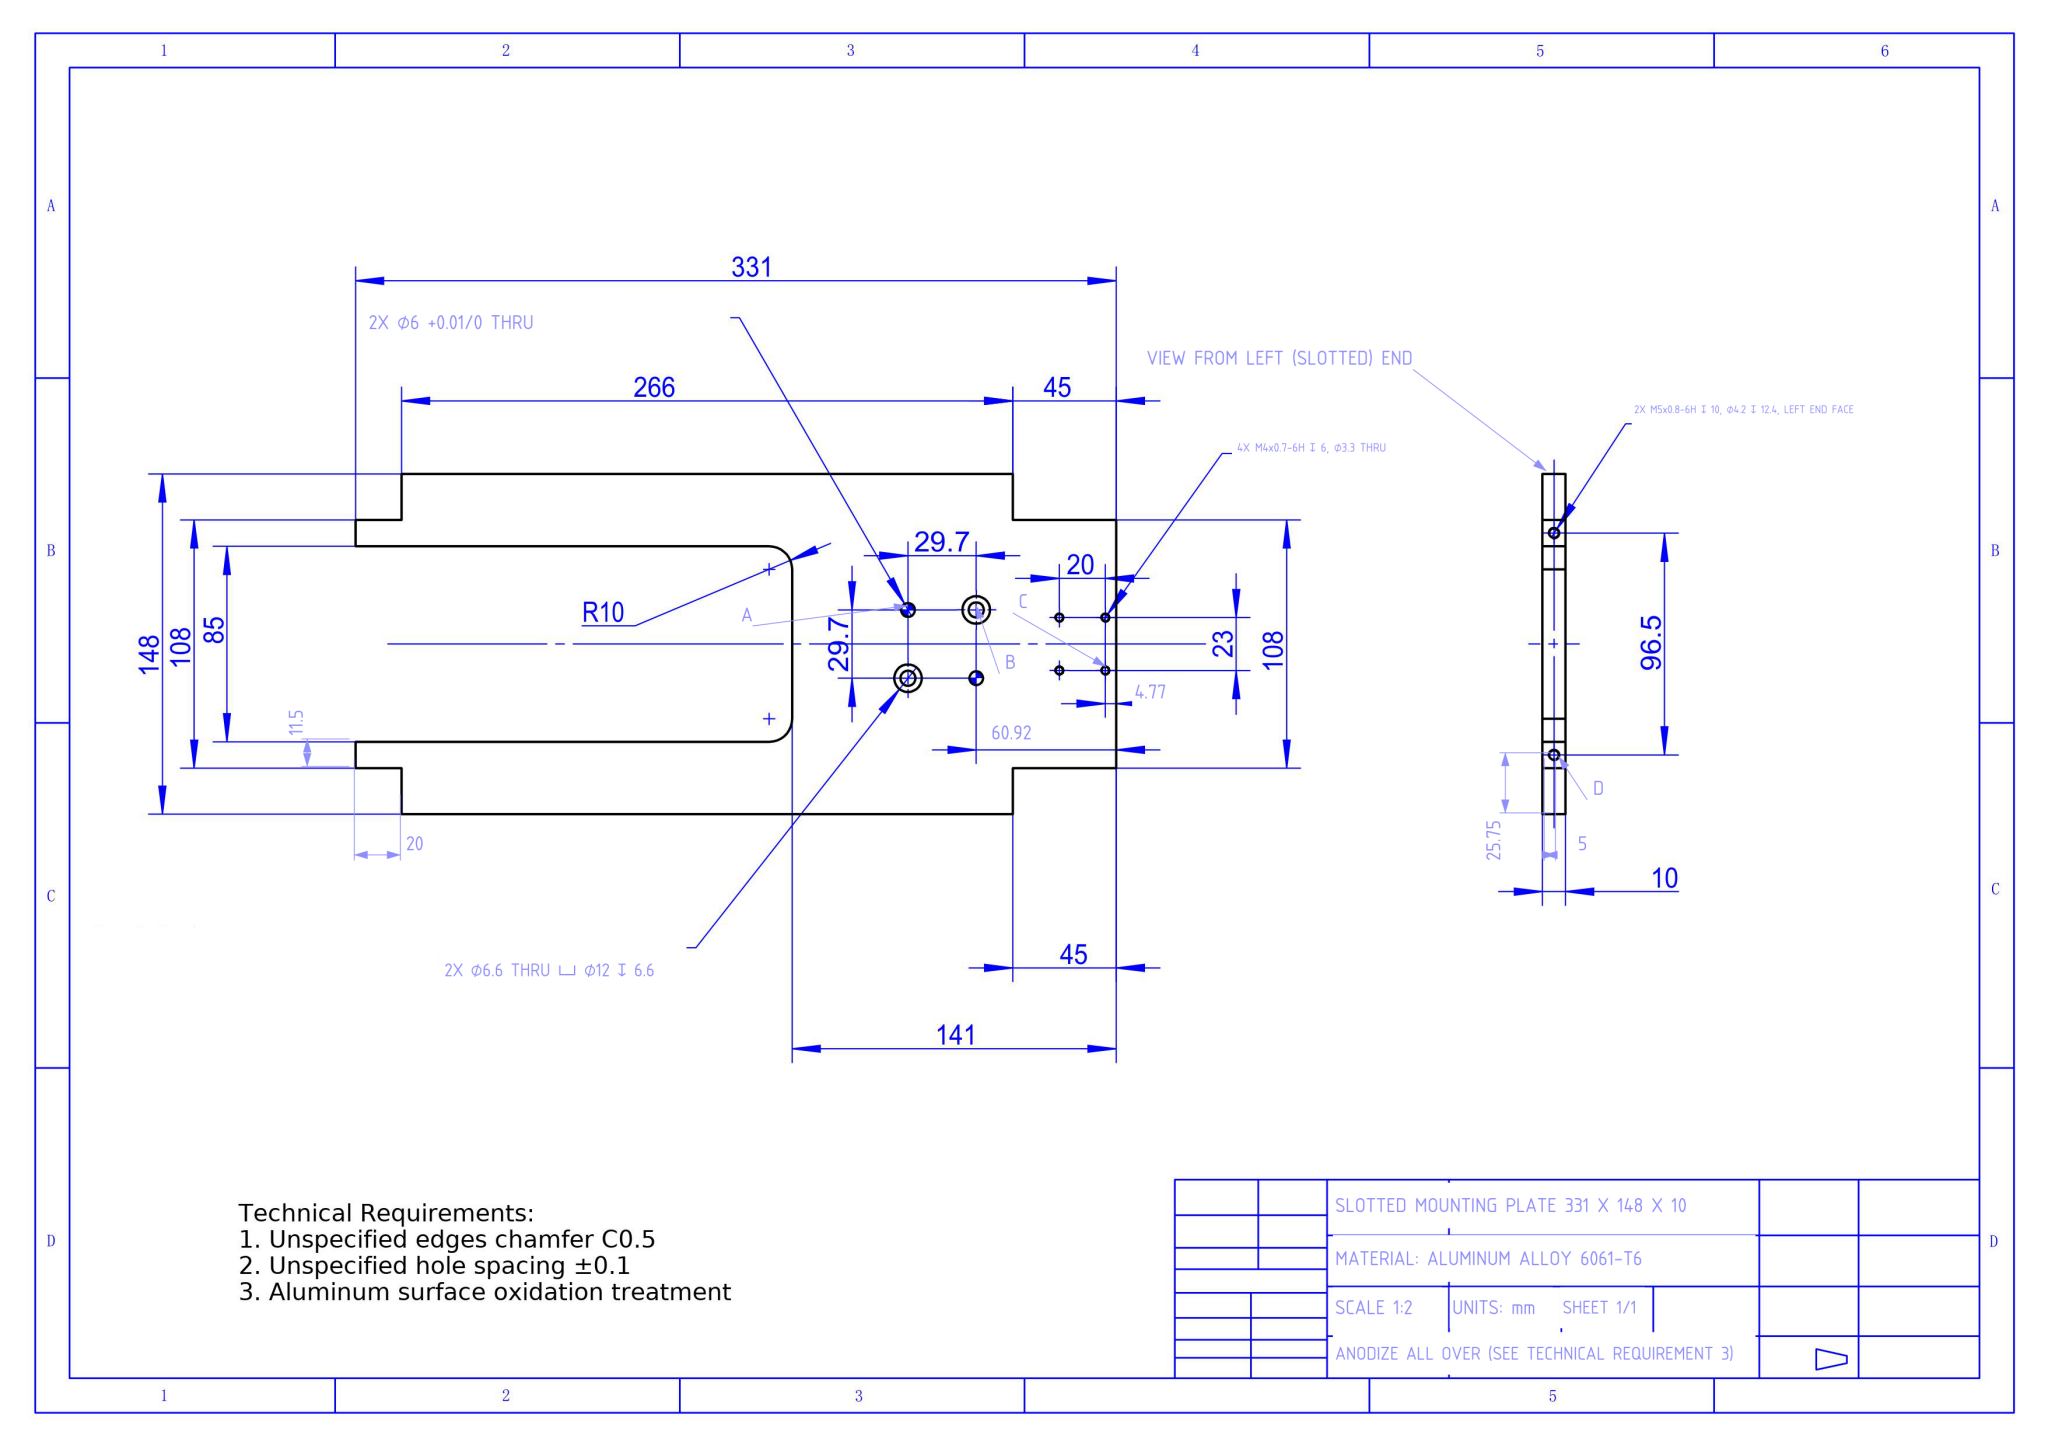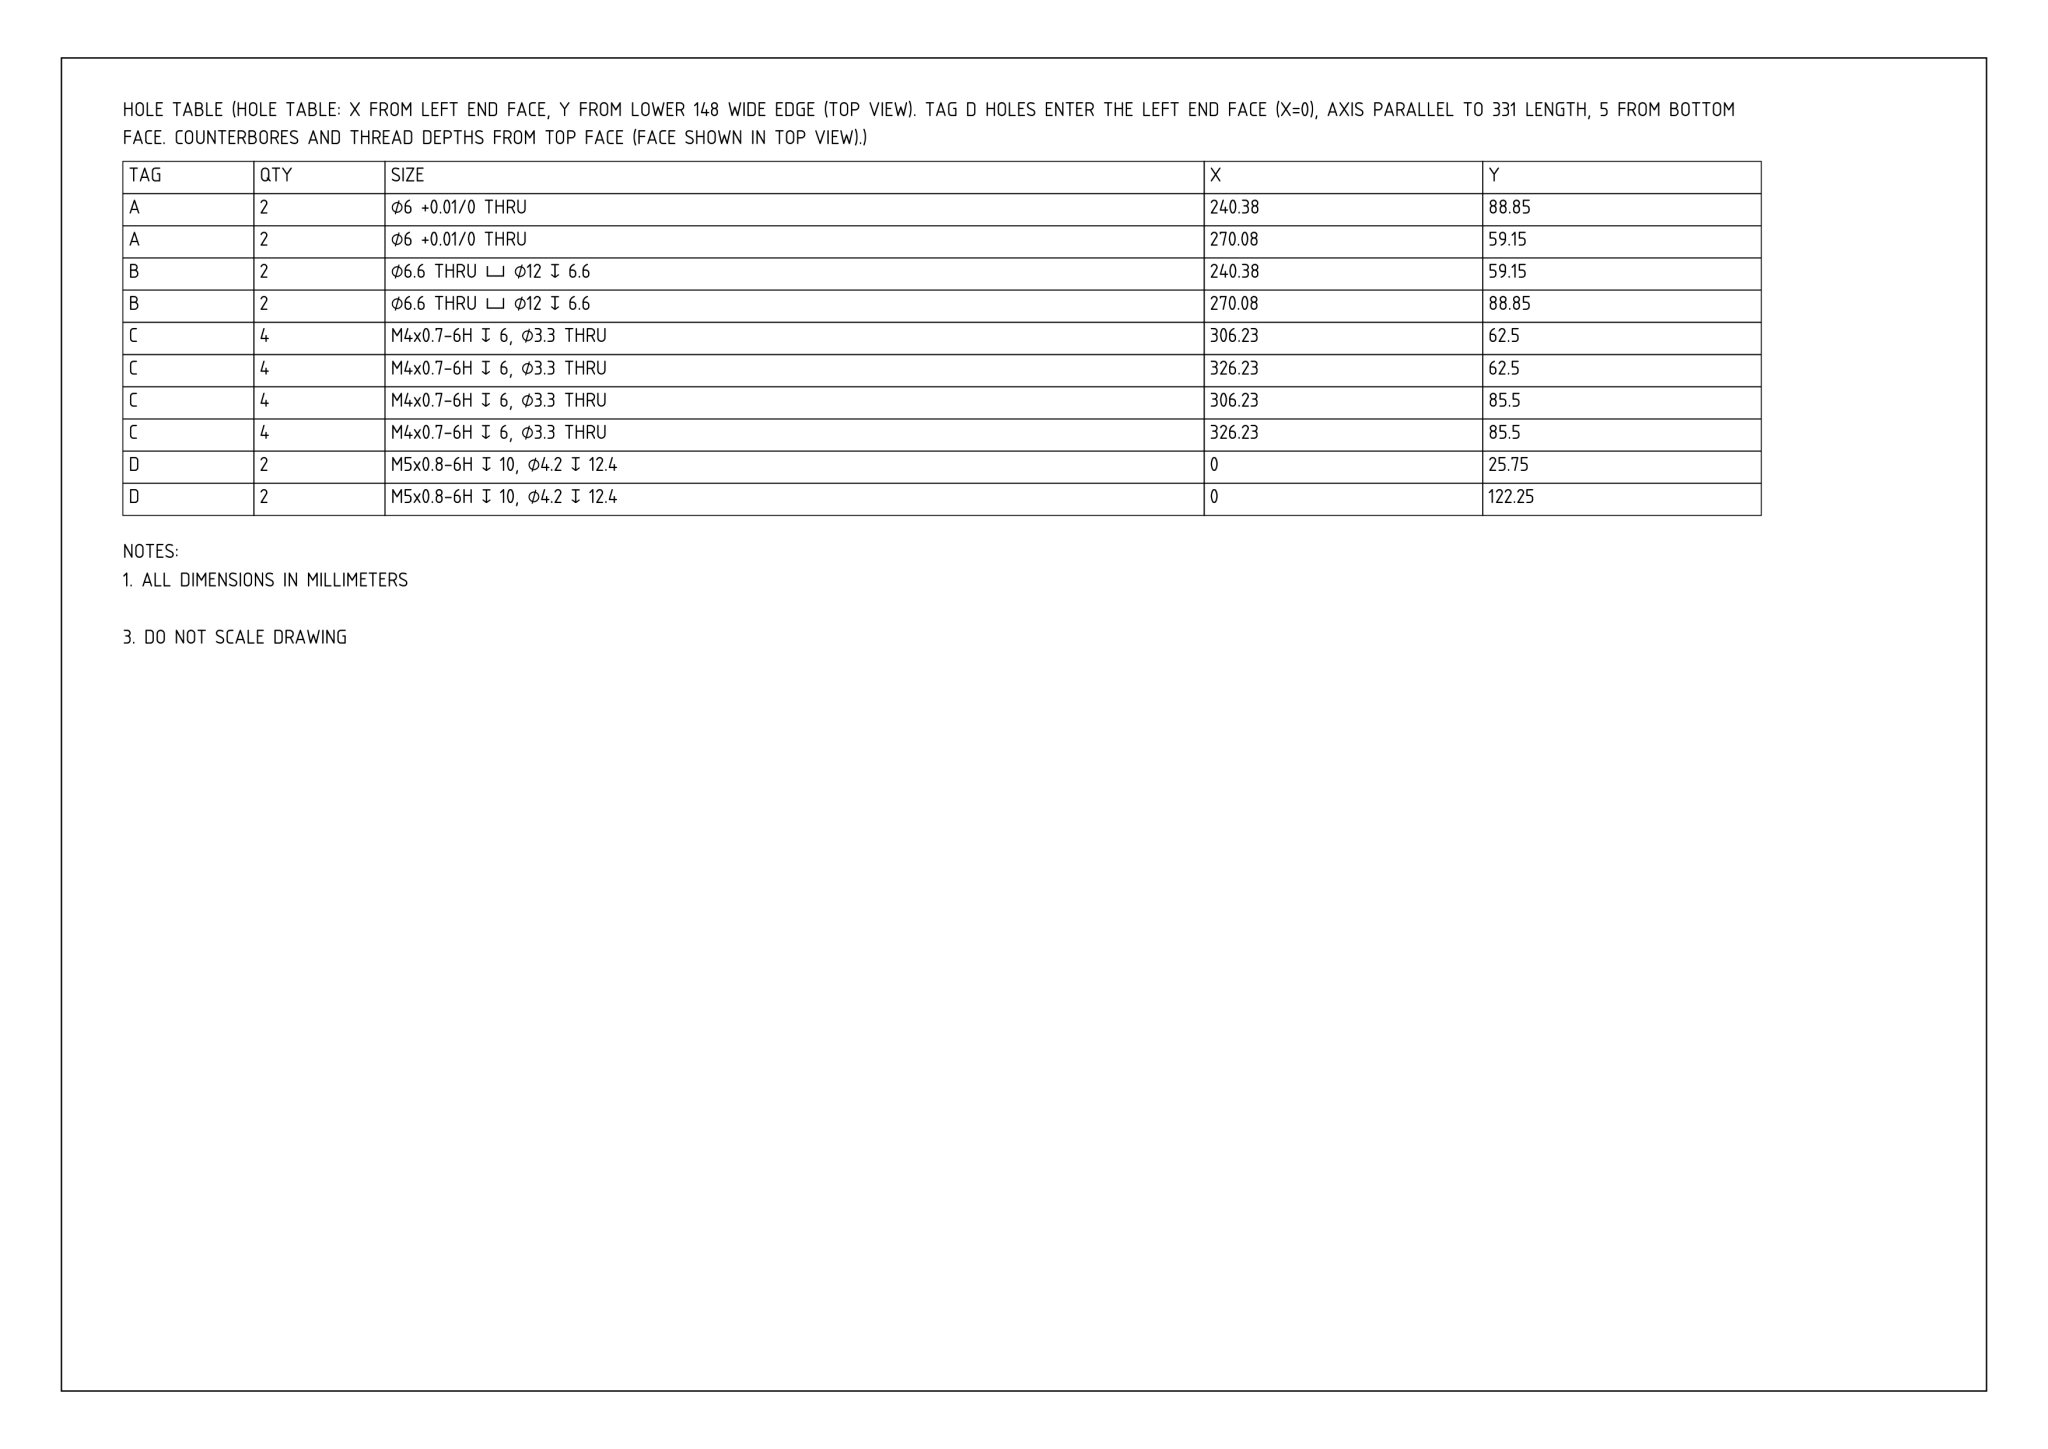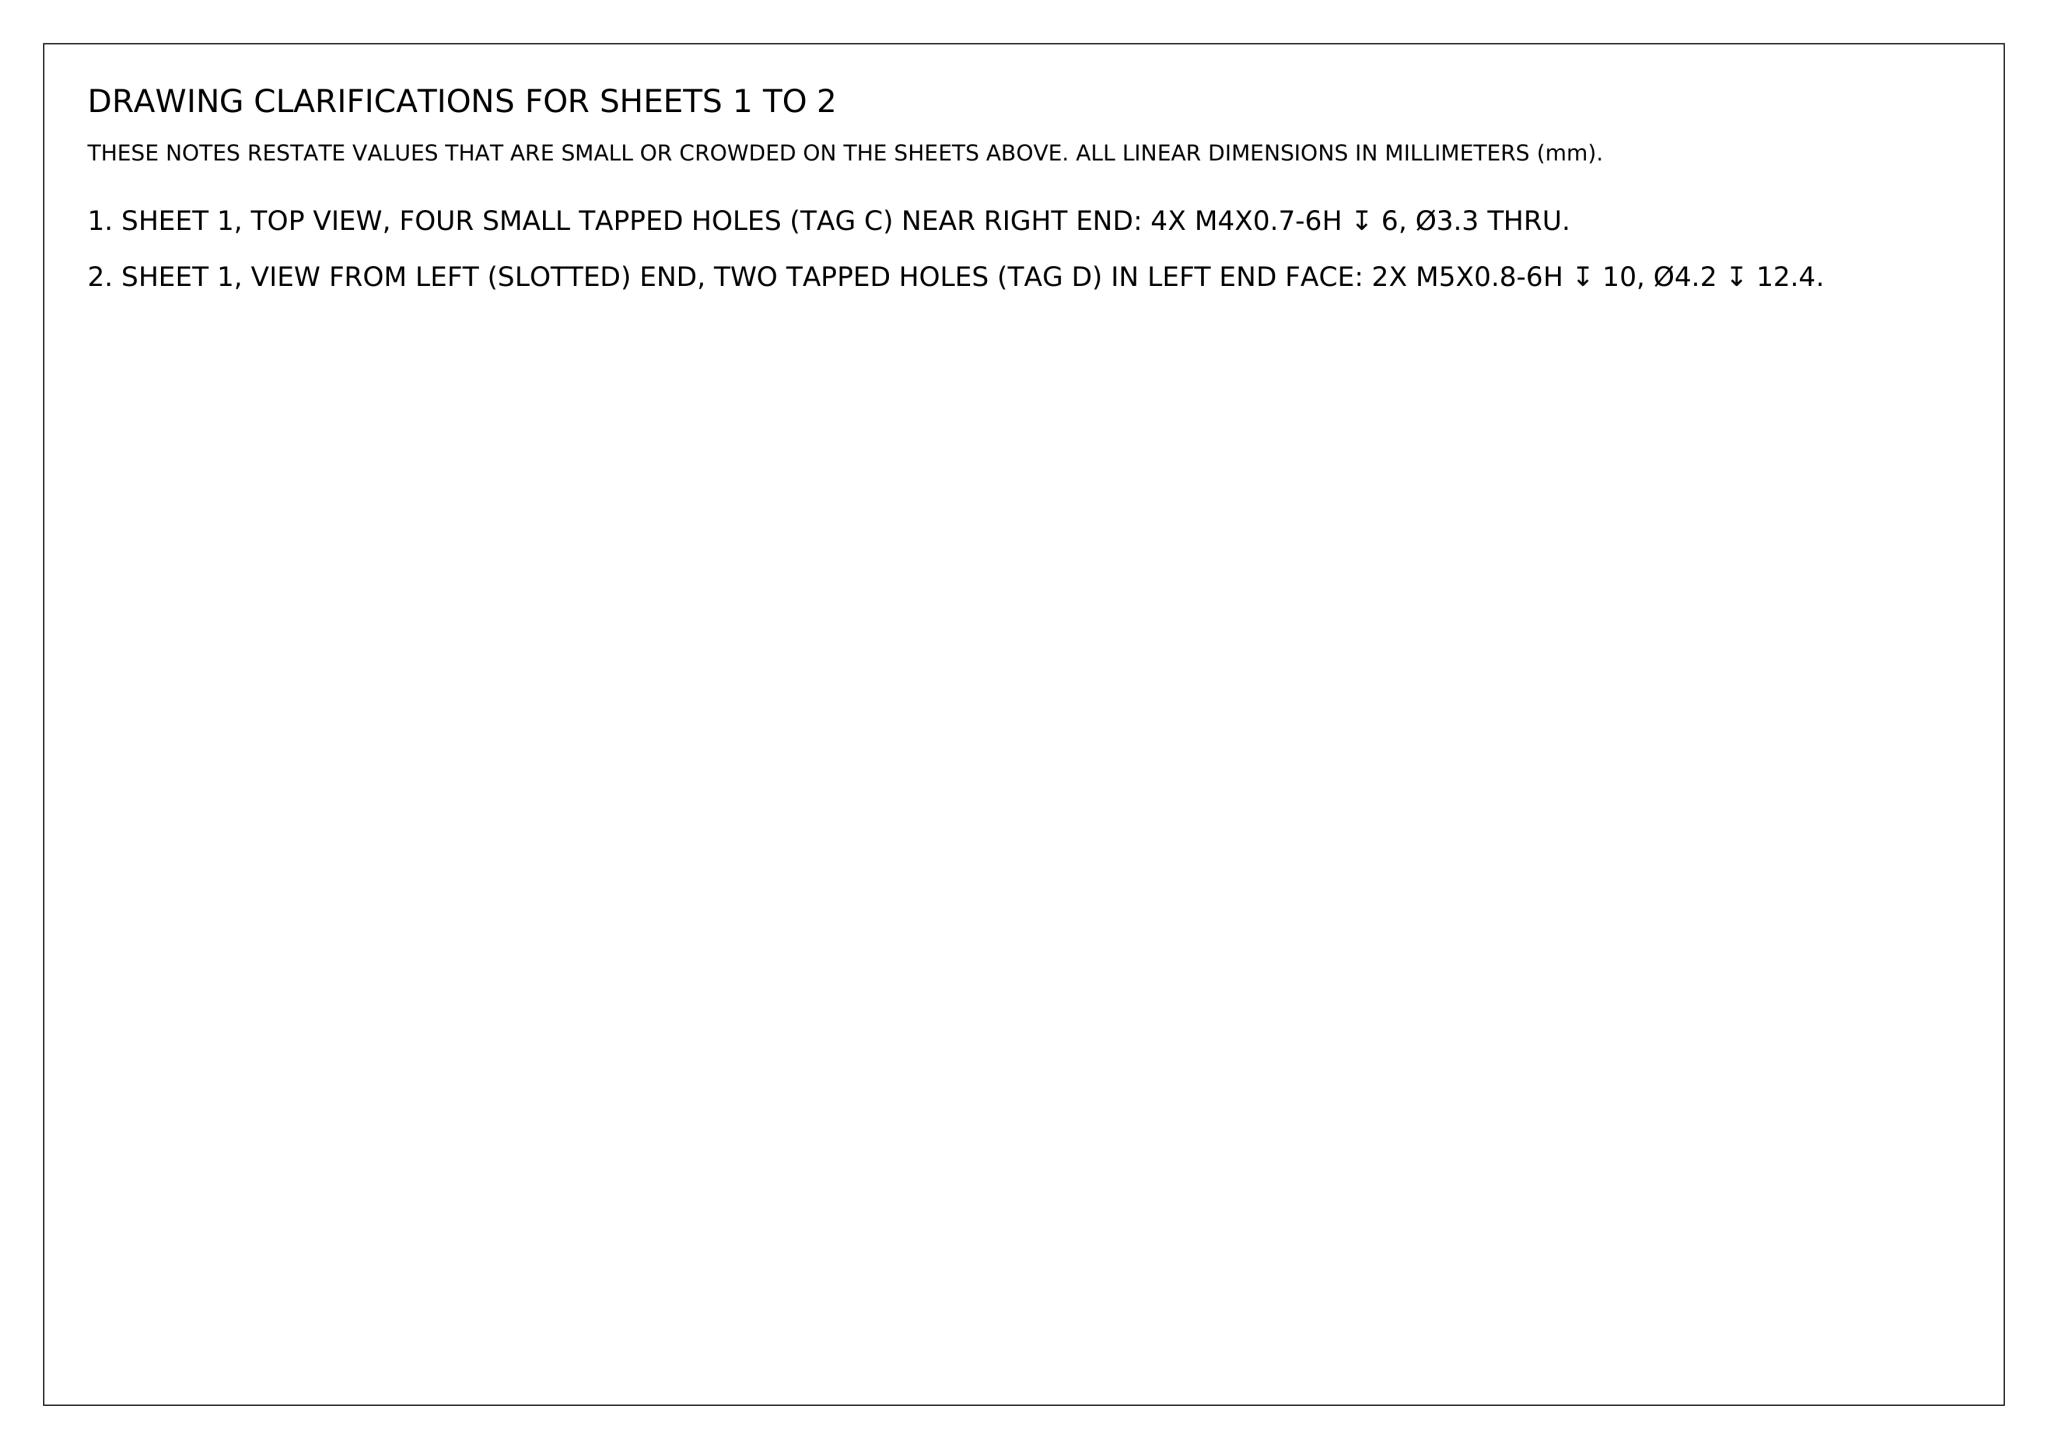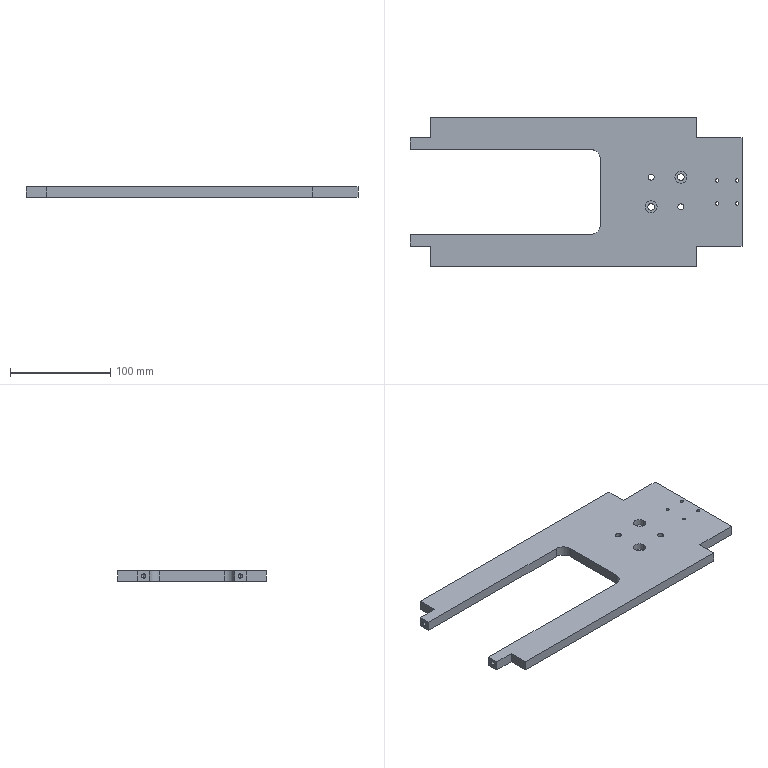Part | NX | mm | 1 solid | 50 faces | box 331 x 148 x 10 mm | volume 299821 mm3 | cylinder 26 | plane 20 | cone 4 | commonest cylinder face diameters 3.3 x8 4.2 x4 6 x4 12 x4 6.6 x4 20 x2